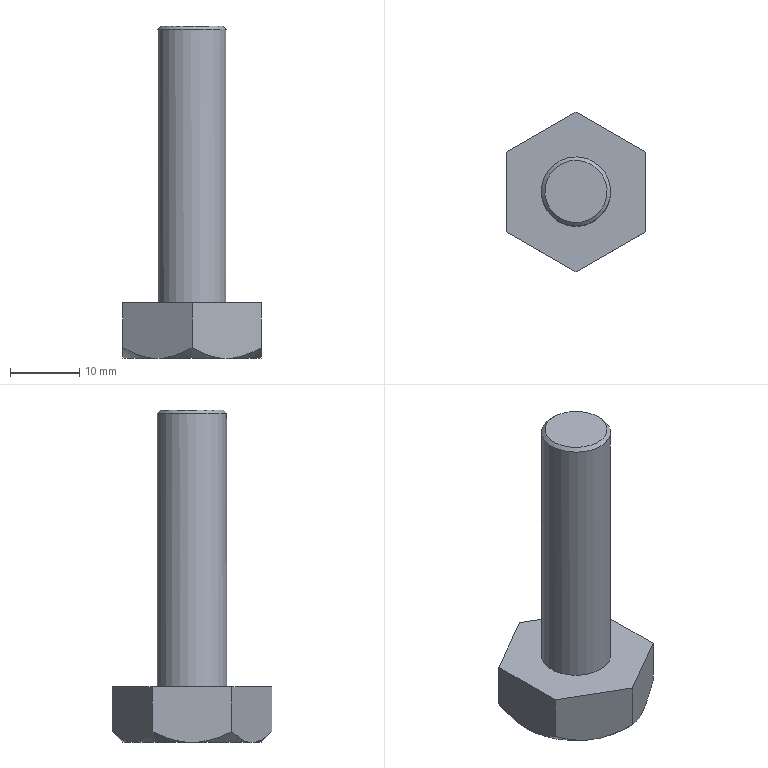Component | NX | HEXSCREWM10_2 | 1 solid | 17 faces | volume 5895 mm3 | plane 9 | cone 7 | cylinder 1 | commonest cylinder face diameters 10 x1